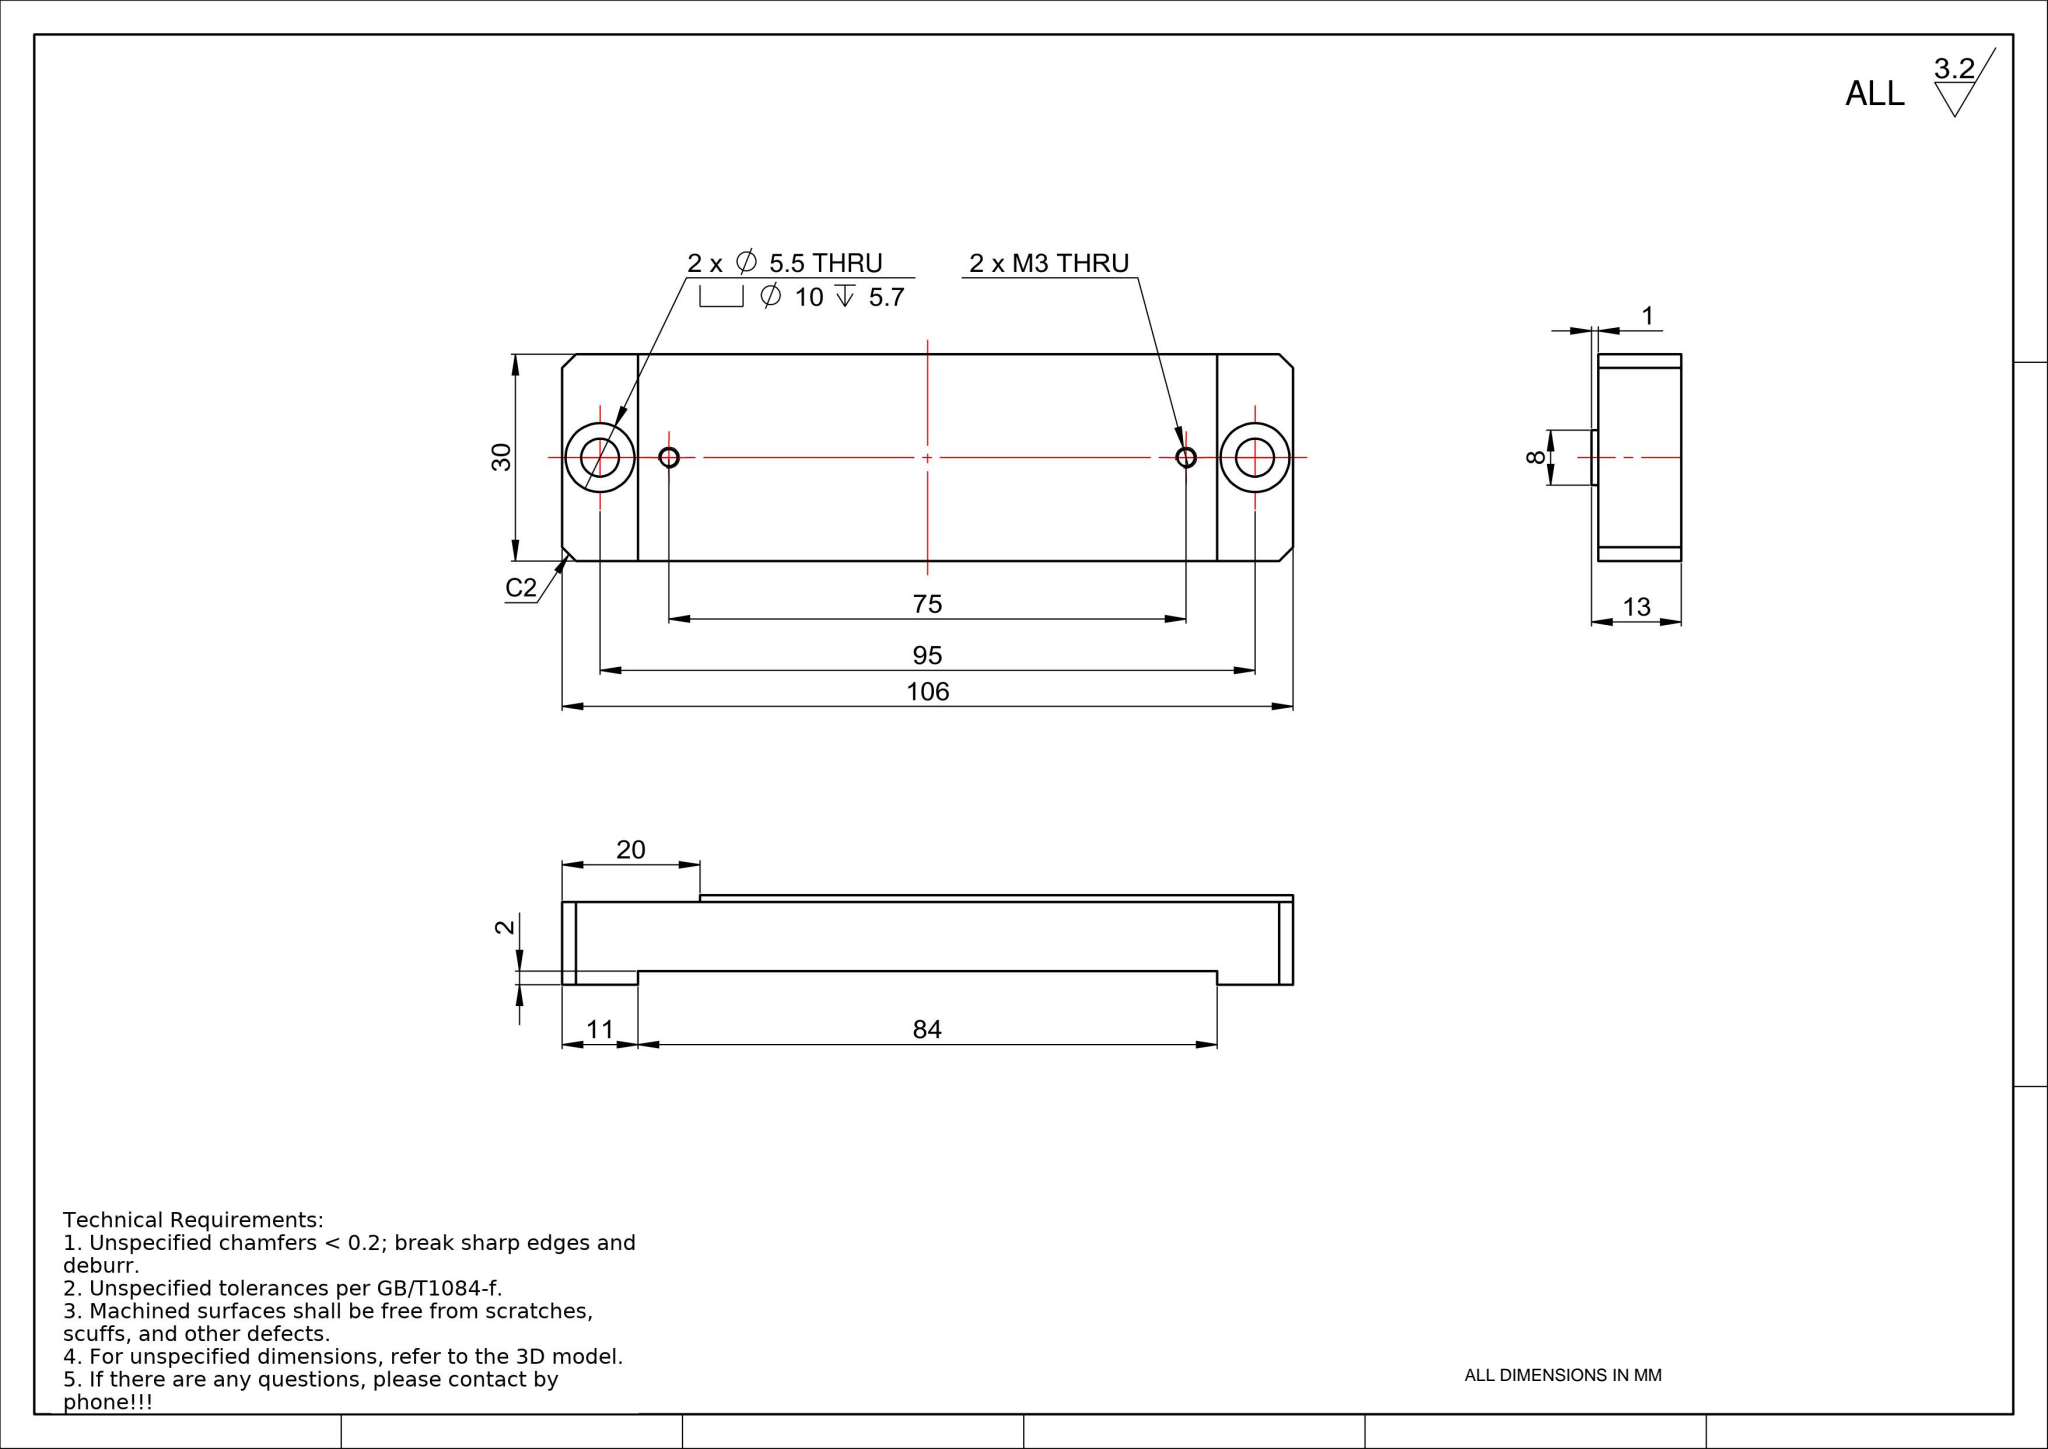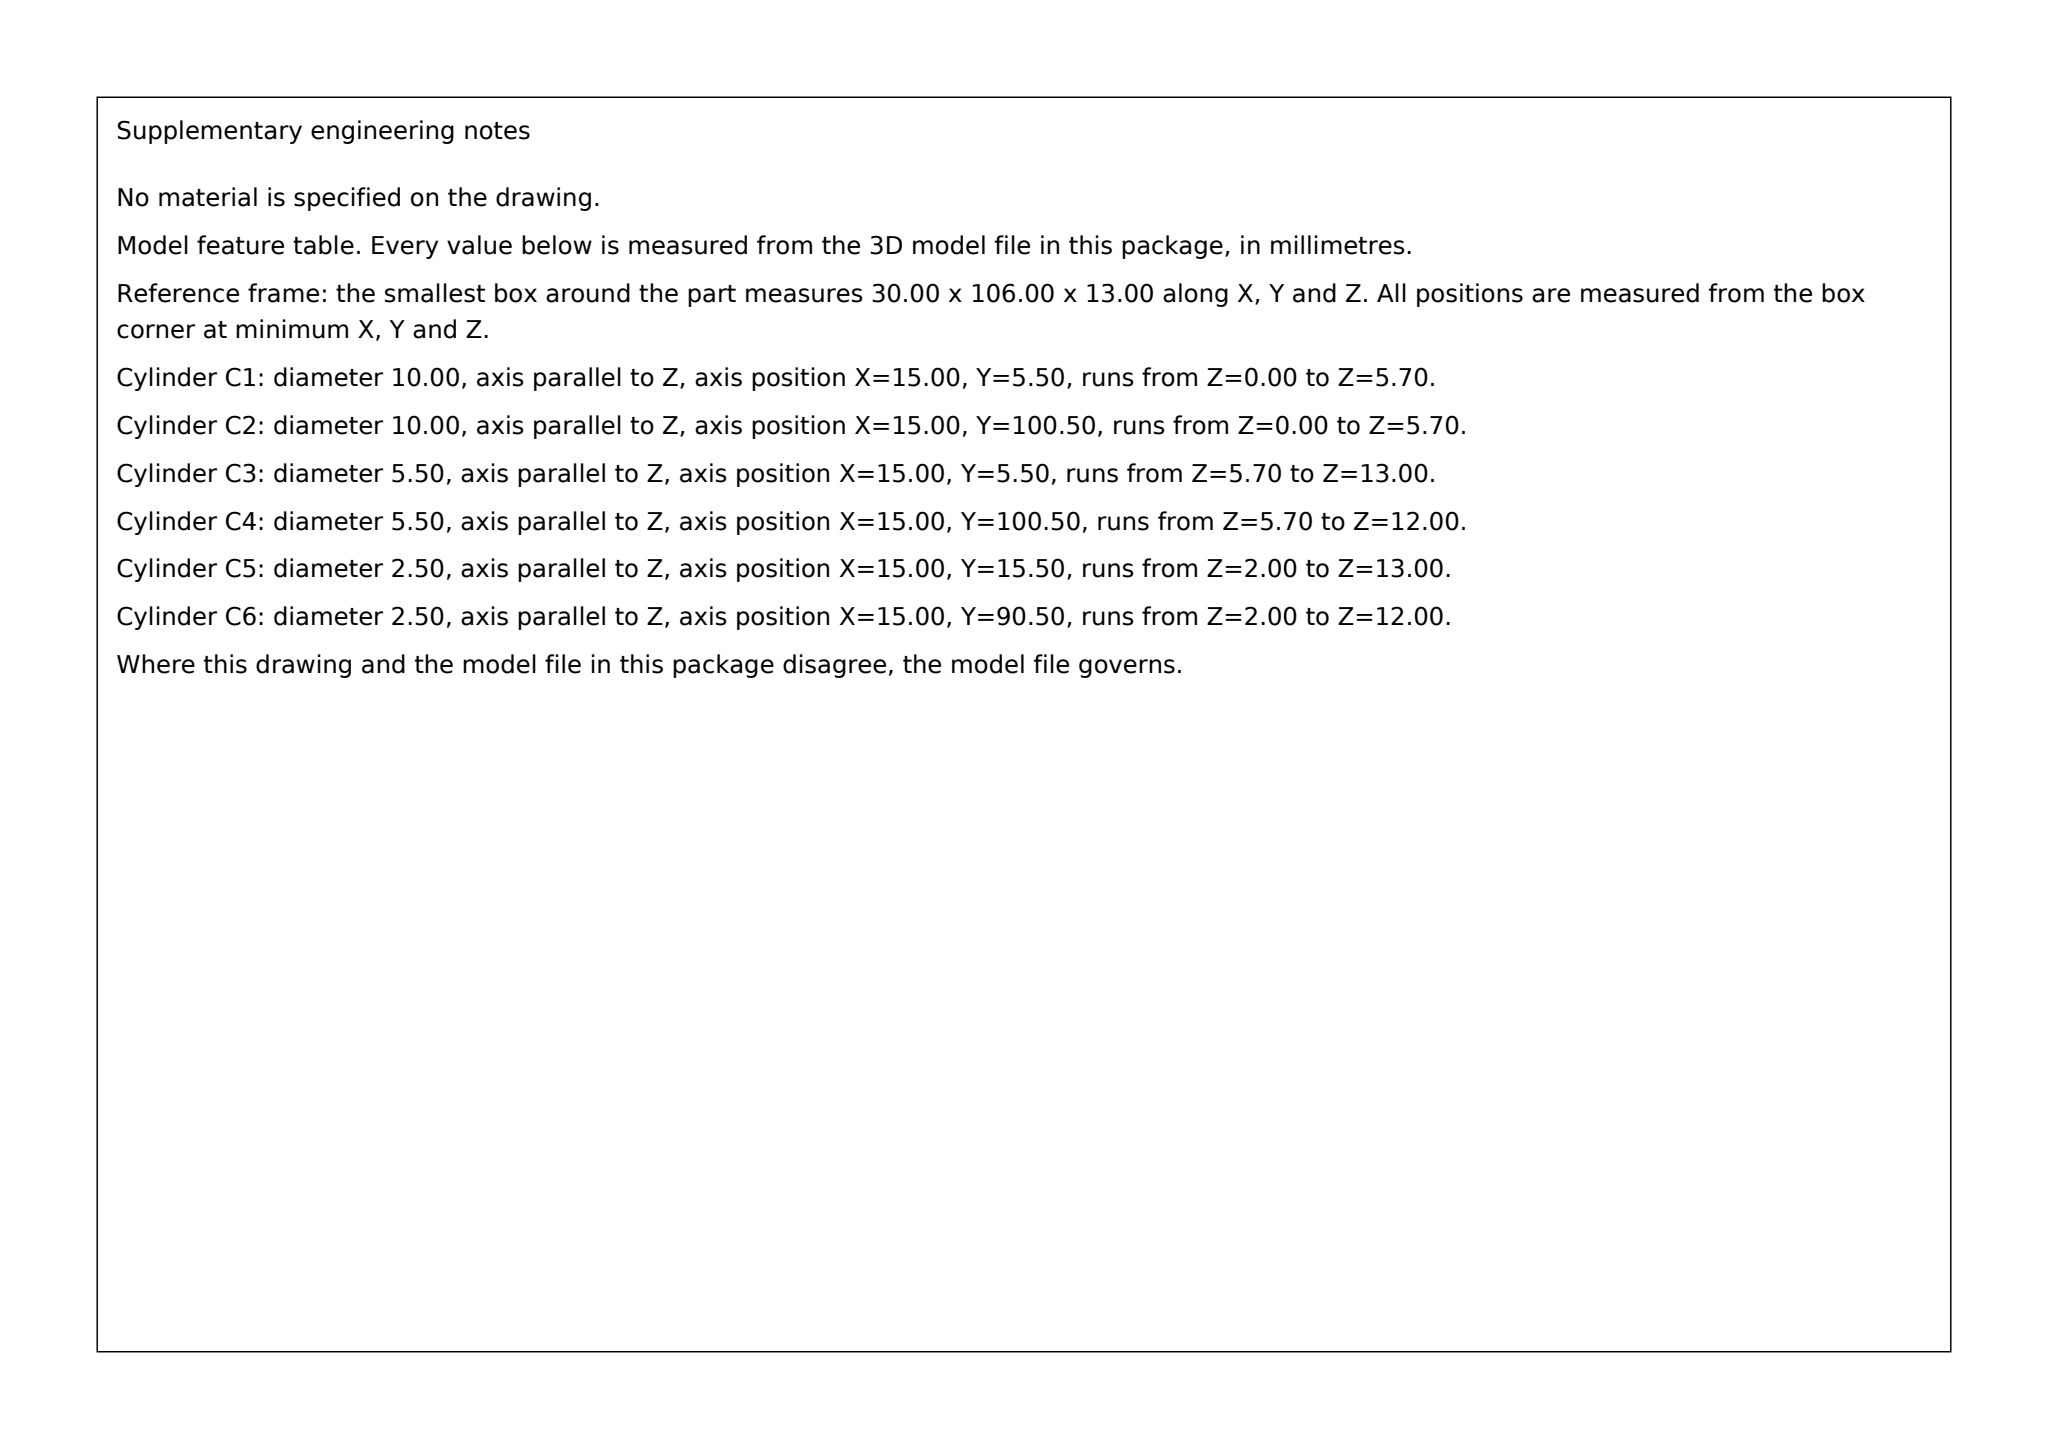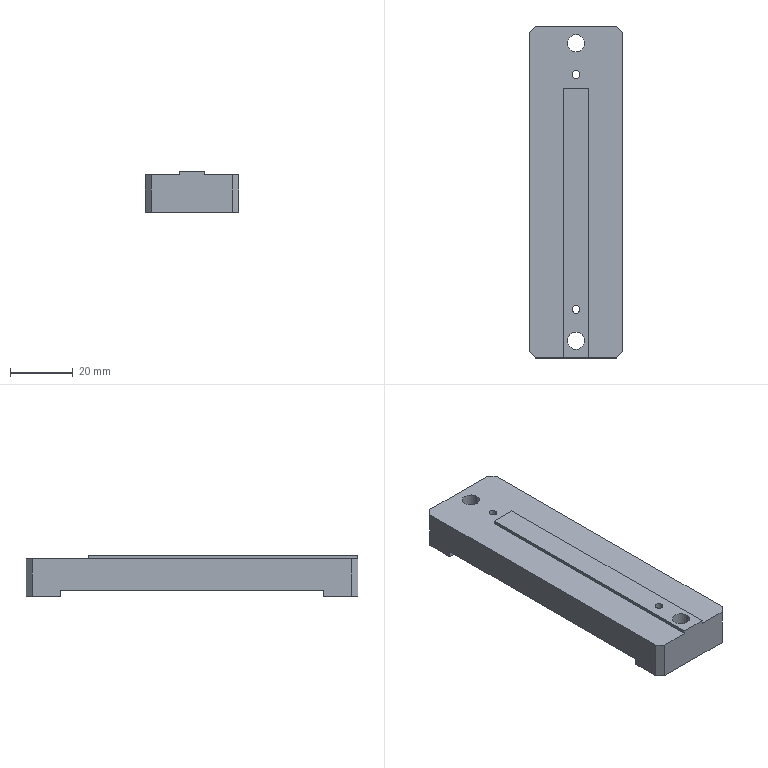Part | SolidWorks | mm | 1 solid | 32 faces | box 30 x 106 x 13 mm | volume 32390 mm3 | plane 20 | cylinder 12 | commonest cylinder face diameters 2.5 x4 10 x4 5.5 x4
build123d program:
from build123d import *

# Parameters (mm, degrees)
SKETCH1_W                                         = 30
SKETCH1_H                                         = 106
BOSS_EXTRUDE1_DEPTH                               = 13
CUT_EXTRUDE1_DEPTH                                = 1
SKETCH3_W                                         = 30
SKETCH3_H                                         = 84
CUT_EXTRUDE2_DEPTH                                = 2
CHAMFER1_SIZE                                     = 2
HOLE_SIZE_ACCORDING_TO_HEX_SOCKET_HEA_D           = 5.5
HOLE_SIZE_ACCORDING_TO_HEX_SOCKET_HEA_CBORE_D     = 10
HOLE_SIZE_ACCORDING_TO_HEX_SOCKET_HEA_CBORE_DEPTH = 5.7
M3_TAPPED_HOLE1_D                                 = 2.5


with BuildPart() as part:
    # Sketch1 → Boss-Extrude1 (new body)
    with BuildSketch(Plane.XY):
        with Locations((0, 53)):
            Rectangle(SKETCH1_W, SKETCH1_H)
    extrude(amount=BOSS_EXTRUDE1_DEPTH)

    # Sketch2 → Cut-Extrude1 (cut)
    with BuildSketch(Plane.XY.offset(13)):
        Polygon((4, 0), (4, 86), (-4, 86), (-4, 0), (-15, 0), (-15, 106), (-4, 106), (4, 106), (15, 106), (15, 0), align=None)
    extrude(amount=-CUT_EXTRUDE1_DEPTH, mode=Mode.SUBTRACT)

    # Sketch3 → Cut-Extrude2 (cut)
    with BuildSketch(Plane(origin=(0, 0, 0), x_dir=(-1, 0, 0), z_dir=(0, 0, -1))):
        with Locations((0, 53)):
            Rectangle(SKETCH3_W, SKETCH3_H)
    extrude(amount=-CUT_EXTRUDE2_DEPTH, mode=Mode.SUBTRACT)

    # Chamfer1
    chamfer1_edges = [part.edges().sort_by_distance(p)[0] for p in [
        (-15, 106, 6),
        (15, 106, 6),
        (15, 0, 6),
        (-15, 0, 6),
    ]]
    chamfer(chamfer1_edges, length=CHAMFER1_SIZE)

    # Hole Size _ according to_ Hex Socket Hea (through all)
    with Locations(Plane(origin=(0, 0, 0), x_dir=(-1, 0, 0), z_dir=(0, 0, -1))):
        with Locations((0, 5.5), (0, 100.5)):
            CounterBoreHole(HOLE_SIZE_ACCORDING_TO_HEX_SOCKET_HEA_D / 2, HOLE_SIZE_ACCORDING_TO_HEX_SOCKET_HEA_CBORE_D / 2, HOLE_SIZE_ACCORDING_TO_HEX_SOCKET_HEA_CBORE_DEPTH)

    # M3 Tapped Hole1 (through all)
    with Locations(Plane(origin=(0, 0, 2), x_dir=(-1, 0, 0), z_dir=(0, 0, -1))):
        with Locations((0, 90.5), (0, 15.5)):
            Hole(M3_TAPPED_HOLE1_D / 2)


solid = part.part